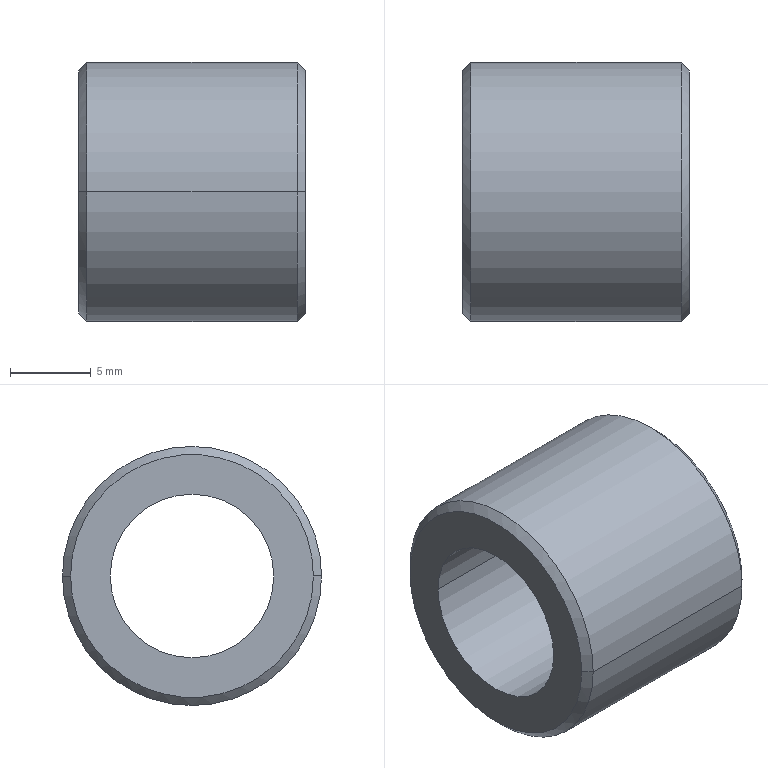Component | SolidWorks | ClampingArm2-1_A75-1 | 1 solid | 10 faces | box 14 x 16 x 16 mm | volume 1681 mm3 | cone 4 | cylinder 4 | plane 2 | commonest cylinder face diameters 10.1 x2 16 x2 | material Brass
build123d program:
from build123d import *

# Parameters (mm, degrees)
SKETCH1_R           = 8
SKETCH1_R_2         = 5.05
BOSS_EXTRUDE1_DEPTH = 7
CHAMFER1_SIZE       = 0.5


with BuildPart() as part:
    # Sketch1 → Boss-Extrude1 (new, symmetric)
    with BuildSketch(Plane(origin=(0, 0, 0), x_dir=(0, 0, -1), z_dir=(1, 0, 0))):
        Circle(SKETCH1_R)
        Circle(SKETCH1_R_2, mode=Mode.SUBTRACT)
    extrude(amount=BOSS_EXTRUDE1_DEPTH, both=True)

    # Chamfer1
    chamfer1_edges = [part.edges().sort_by_distance(p)[0] for p in [
        (-7, 0, 8),
        (7, 0, 8),
    ]]
    chamfer(chamfer1_edges, length=CHAMFER1_SIZE)


solid = part.part

# Placed as in the assembly
solid = solid.moved(Location((-22.051, 66.046, -22.5), (0, 0, 0)))
STEP:
#1=CARTESIAN_POINT('',(-0.5925,2.896,-0.8859));
#2=VERTEX_POINT('',#1);
#3=CARTESIAN_POINT('',(-0.5925,2.305,-0.8857));
#4=VERTEX_POINT('',#3);
#5=CARTESIAN_POINT('',(-0.5925,2.6,-0.8858));
#6=DIRECTION('',(1.,0.,-0.));
#7=DIRECTION('',(-0.,1.,-0.0003333));
#8=AXIS2_PLACEMENT_3D('',#5,#6,#7);
#9=CIRCLE('',#8,0.2953);
#10=EDGE_CURVE('',#2,#4,#9,.T.);
#11=ORIENTED_EDGE('',*,*,#10,.F.);
#12=CARTESIAN_POINT('',(-0.6122,2.915,-0.8859));
#13=VERTEX_POINT('',#12);
#14=CARTESIAN_POINT('',(-0.5925,2.896,-0.8859));
#15=DIRECTION('',(-0.7071,0.7071,-0.0002357));
#16=VECTOR('',#15,39.37);
#17=LINE('',#14,#16);
#18=EDGE_CURVE('',#2,#13,#17,.T.);
#19=ORIENTED_EDGE('',*,*,#18,.T.);
#20=CARTESIAN_POINT('',(-0.6122,2.285,-0.8857));
#21=VERTEX_POINT('',#20);
#22=CARTESIAN_POINT('',(-0.6122,2.6,-0.8858));
#23=DIRECTION('',(-1.,-0.,0.));
#24=DIRECTION('',(-0.,1.,-0.0003333));
#25=AXIS2_PLACEMENT_3D('',#22,#23,#24);
#26=CIRCLE('',#25,0.315);
#27=EDGE_CURVE('',#21,#13,#26,.T.);
#28=ORIENTED_EDGE('',*,*,#27,.F.);
#29=CARTESIAN_POINT('',(-0.5925,2.305,-0.8857));
#30=DIRECTION('',(-0.7071,-0.7071,0.0002357));
#31=VECTOR('',#30,39.37);
#32=LINE('',#29,#31);
#33=EDGE_CURVE('',#4,#21,#32,.T.);
#34=ORIENTED_EDGE('',*,*,#33,.F.);
#35=EDGE_LOOP('',(#11,#19,#28,#34));
#36=FACE_OUTER_BOUND('',#35,.T.);
#37=CARTESIAN_POINT('',(-0.5925,2.6,-0.8858));
#38=DIRECTION('',(-1.,-0.,0.));
#39=DIRECTION('',(0.,-1.,0.0003333));
#40=AXIS2_PLACEMENT_3D('',#37,#38,#39);
#41=CONICAL_SURFACE('',#40,0.2953,0.7854);
#42=ADVANCED_FACE('',(#36),#41,.T.);
#43=CARTESIAN_POINT('',(-1.144,2.305,-0.8857));
#44=VERTEX_POINT('',#43);
#45=CARTESIAN_POINT('',(-1.144,2.896,-0.8859));
#46=VERTEX_POINT('',#45);
#47=CARTESIAN_POINT('',(-1.144,2.6,-0.8858));
#48=DIRECTION('',(-1.,-0.,0.));
#49=DIRECTION('',(-0.,1.,-0.0003333));
#50=AXIS2_PLACEMENT_3D('',#47,#48,#49);
#51=CIRCLE('',#50,0.2953);
#52=EDGE_CURVE('',#44,#46,#51,.T.);
#53=ORIENTED_EDGE('',*,*,#52,.F.);
#54=CARTESIAN_POINT('',(-1.124,2.285,-0.8857));
#55=VERTEX_POINT('',#54);
#56=CARTESIAN_POINT('',(-1.124,2.285,-0.8857));
#57=DIRECTION('',(0.7071,-0.7071,0.0002357));
#58=VECTOR('',#57,39.37);
#59=LINE('',#56,#58);
#60=EDGE_CURVE('',#44,#55,#59,.T.);
#61=ORIENTED_EDGE('',*,*,#60,.T.);
#62=CARTESIAN_POINT('',(-1.124,2.915,-0.8859));
#63=VERTEX_POINT('',#62);
#64=CARTESIAN_POINT('',(-1.124,2.6,-0.8858));
#65=DIRECTION('',(1.,0.,-0.));
#66=DIRECTION('',(-0.,1.,-0.0003333));
#67=AXIS2_PLACEMENT_3D('',#64,#65,#66);
#68=CIRCLE('',#67,0.315);
#69=EDGE_CURVE('',#63,#55,#68,.T.);
#70=ORIENTED_EDGE('',*,*,#69,.F.);
#71=CARTESIAN_POINT('',(-1.124,2.915,-0.8859));
#72=DIRECTION('',(0.7071,0.7071,-0.0002357));
#73=VECTOR('',#72,39.37);
#74=LINE('',#71,#73);
#75=EDGE_CURVE('',#46,#63,#74,.T.);
#76=ORIENTED_EDGE('',*,*,#75,.F.);
#77=EDGE_LOOP('',(#53,#61,#70,#76));
#78=FACE_OUTER_BOUND('',#77,.T.);
#79=CARTESIAN_POINT('',(-1.124,2.6,-0.8858));
#80=DIRECTION('',(1.,0.,-0.));
#81=DIRECTION('',(-0.,1.,-0.0003333));
#82=AXIS2_PLACEMENT_3D('',#79,#80,#81);
#83=CONICAL_SURFACE('',#82,0.315,0.7854);
#84=ADVANCED_FACE('',(#78),#83,.T.);
#85=CARTESIAN_POINT('',(-0.5925,2.401,-0.8858));
#86=VERTEX_POINT('',#85);
#87=CARTESIAN_POINT('',(-0.5925,2.799,-0.8859));
#88=VERTEX_POINT('',#87);
#89=CARTESIAN_POINT('',(-0.5925,2.6,-0.8858));
#90=DIRECTION('',(1.,0.,-0.));
#91=DIRECTION('',(-0.,1.,-0.0003333));
#92=AXIS2_PLACEMENT_3D('',#89,#90,#91);
#93=CIRCLE('',#92,0.1988);
#94=EDGE_CURVE('',#86,#88,#93,.T.);
#95=ORIENTED_EDGE('',*,*,#94,.T.);
#96=CARTESIAN_POINT('',(-1.144,2.799,-0.8859));
#97=VERTEX_POINT('',#96);
#98=CARTESIAN_POINT('',(-0.5925,2.799,-0.8859));
#99=DIRECTION('',(-1.,-0.,0.));
#100=VECTOR('',#99,39.37);
#101=LINE('',#98,#100);
#102=EDGE_CURVE('',#88,#97,#101,.T.);
#103=ORIENTED_EDGE('',*,*,#102,.T.);
#104=CARTESIAN_POINT('',(-1.144,2.401,-0.8858));
#105=VERTEX_POINT('',#104);
#106=CARTESIAN_POINT('',(-1.144,2.6,-0.8858));
#107=DIRECTION('',(1.,0.,-0.));
#108=DIRECTION('',(0.,1.,-0.0003333));
#109=AXIS2_PLACEMENT_3D('',#106,#107,#108);
#110=CIRCLE('',#109,0.1988);
#111=EDGE_CURVE('',#105,#97,#110,.T.);
#112=ORIENTED_EDGE('',*,*,#111,.F.);
#113=CARTESIAN_POINT('',(-0.5925,2.401,-0.8858));
#114=DIRECTION('',(-1.,-0.,0.));
#115=VECTOR('',#114,39.37);
#116=LINE('',#113,#115);
#117=EDGE_CURVE('',#86,#105,#116,.T.);
#118=ORIENTED_EDGE('',*,*,#117,.F.);
#119=EDGE_LOOP('',(#95,#103,#112,#118));
#120=FACE_OUTER_BOUND('',#119,.T.);
#121=CARTESIAN_POINT('',(-0.5925,2.6,-0.8858));
#122=DIRECTION('',(-1.,-0.,0.));
#123=DIRECTION('',(0.,-1.,0.0003333));
#124=AXIS2_PLACEMENT_3D('',#121,#122,#123);
#125=CYLINDRICAL_SURFACE('',#124,0.1988);
#126=ADVANCED_FACE('',(#120),#125,.F.);
#127=ORIENTED_EDGE('',*,*,#27,.T.);
#128=CARTESIAN_POINT('',(-0.5925,2.915,-0.8859));
#129=DIRECTION('',(-1.,-0.,0.));
#130=VECTOR('',#129,39.37);
#131=LINE('',#128,#130);
#132=EDGE_CURVE('',#13,#63,#131,.T.);
#133=ORIENTED_EDGE('',*,*,#132,.T.);
#134=ORIENTED_EDGE('',*,*,#69,.T.);
#135=CARTESIAN_POINT('',(-0.5925,2.285,-0.8857));
#136=DIRECTION('',(-1.,-0.,0.));
#137=VECTOR('',#136,39.37);
#138=LINE('',#135,#137);
#139=EDGE_CURVE('',#21,#55,#138,.T.);
#140=ORIENTED_EDGE('',*,*,#139,.F.);
#141=EDGE_LOOP('',(#127,#133,#134,#140));
#142=FACE_OUTER_BOUND('',#141,.T.);
#143=CARTESIAN_POINT('',(-0.5925,2.6,-0.8858));
#144=DIRECTION('',(-1.,-0.,0.));
#145=DIRECTION('',(0.,-1.,0.0003333));
#146=AXIS2_PLACEMENT_3D('',#143,#144,#145);
#147=CYLINDRICAL_SURFACE('',#146,0.315);
#148=ADVANCED_FACE('',(#142),#147,.T.);
#149=CARTESIAN_POINT('',(-0.5925,2.6,-0.8858));
#150=DIRECTION('',(1.,0.,-0.));
#151=DIRECTION('',(-0.,1.,-0.0003333));
#152=AXIS2_PLACEMENT_3D('',#149,#150,#151);
#153=CIRCLE('',#152,0.2953);
#154=EDGE_CURVE('',#4,#2,#153,.T.);
#155=ORIENTED_EDGE('',*,*,#154,.T.);
#156=ORIENTED_EDGE('',*,*,#10,.T.);
#157=EDGE_LOOP('',(#155,#156));
#158=FACE_OUTER_BOUND('',#157,.T.);
#159=ORIENTED_EDGE('',*,*,#94,.F.);
#160=CARTESIAN_POINT('',(-0.5925,2.6,-0.8858));
#161=DIRECTION('',(1.,0.,-0.));
#162=DIRECTION('',(-0.,1.,-0.0003333));
#163=AXIS2_PLACEMENT_3D('',#160,#161,#162);
#164=CIRCLE('',#163,0.1988);
#165=EDGE_CURVE('',#88,#86,#164,.T.);
#166=ORIENTED_EDGE('',*,*,#165,.F.);
#167=EDGE_LOOP('',(#159,#166));
#168=FACE_BOUND('',#167,.T.);
#169=CARTESIAN_POINT('',(-0.5925,2.6,-0.8858));
#170=DIRECTION('',(1.,0.,-0.));
#171=DIRECTION('',(-0.,1.,-0.0003333));
#172=AXIS2_PLACEMENT_3D('',#169,#170,#171);
#173=PLANE('',#172);
#174=ADVANCED_FACE('',(#158,#168),#173,.T.);
#175=CARTESIAN_POINT('',(-1.144,2.6,-0.8858));
#176=DIRECTION('',(-1.,-0.,0.));
#177=DIRECTION('',(-0.,1.,-0.0003333));
#178=AXIS2_PLACEMENT_3D('',#175,#176,#177);
#179=CIRCLE('',#178,0.2953);
#180=EDGE_CURVE('',#46,#44,#179,.T.);
#181=ORIENTED_EDGE('',*,*,#180,.T.);
#182=ORIENTED_EDGE('',*,*,#52,.T.);
#183=EDGE_LOOP('',(#181,#182));
#184=FACE_OUTER_BOUND('',#183,.T.);
#185=ORIENTED_EDGE('',*,*,#111,.T.);
#186=CARTESIAN_POINT('',(-1.144,2.6,-0.8858));
#187=DIRECTION('',(1.,0.,-0.));
#188=DIRECTION('',(0.,1.,-0.0003333));
#189=AXIS2_PLACEMENT_3D('',#186,#187,#188);
#190=CIRCLE('',#189,0.1988);
#191=EDGE_CURVE('',#97,#105,#190,.T.);
#192=ORIENTED_EDGE('',*,*,#191,.T.);
#193=EDGE_LOOP('',(#185,#192));
#194=FACE_BOUND('',#193,.T.);
#195=CARTESIAN_POINT('',(-1.144,2.6,-0.8858));
#196=DIRECTION('',(1.,0.,-0.));
#197=DIRECTION('',(-0.,1.,-0.0003333));
#198=AXIS2_PLACEMENT_3D('',#195,#196,#197);
#199=PLANE('',#198);
#200=ADVANCED_FACE('',(#184,#194),#199,.F.);
#201=ORIENTED_EDGE('',*,*,#132,.F.);
#202=CARTESIAN_POINT('',(-0.6122,2.6,-0.8858));
#203=DIRECTION('',(-1.,-0.,0.));
#204=DIRECTION('',(-0.,1.,-0.0003333));
#205=AXIS2_PLACEMENT_3D('',#202,#203,#204);
#206=CIRCLE('',#205,0.315);
#207=EDGE_CURVE('',#13,#21,#206,.T.);
#208=ORIENTED_EDGE('',*,*,#207,.T.);
#209=ORIENTED_EDGE('',*,*,#139,.T.);
#210=CARTESIAN_POINT('',(-1.124,2.6,-0.8858));
#211=DIRECTION('',(1.,0.,-0.));
#212=DIRECTION('',(-0.,1.,-0.0003333));
#213=AXIS2_PLACEMENT_3D('',#210,#211,#212);
#214=CIRCLE('',#213,0.315);
#215=EDGE_CURVE('',#55,#63,#214,.T.);
#216=ORIENTED_EDGE('',*,*,#215,.T.);
#217=EDGE_LOOP('',(#201,#208,#209,#216));
#218=FACE_OUTER_BOUND('',#217,.T.);
#219=CARTESIAN_POINT('',(-0.5925,2.6,-0.8858));
#220=DIRECTION('',(-1.,-0.,0.));
#221=DIRECTION('',(0.,-1.,0.0003333));
#222=AXIS2_PLACEMENT_3D('',#219,#220,#221);
#223=CYLINDRICAL_SURFACE('',#222,0.315);
#224=ADVANCED_FACE('',(#218),#223,.T.);
#225=ORIENTED_EDGE('',*,*,#102,.F.);
#226=ORIENTED_EDGE('',*,*,#165,.T.);
#227=ORIENTED_EDGE('',*,*,#117,.T.);
#228=ORIENTED_EDGE('',*,*,#191,.F.);
#229=EDGE_LOOP('',(#225,#226,#227,#228));
#230=FACE_OUTER_BOUND('',#229,.T.);
#231=CARTESIAN_POINT('',(-0.5925,2.6,-0.8858));
#232=DIRECTION('',(-1.,-0.,0.));
#233=DIRECTION('',(0.,-1.,0.0003333));
#234=AXIS2_PLACEMENT_3D('',#231,#232,#233);
#235=CYLINDRICAL_SURFACE('',#234,0.1988);
#236=ADVANCED_FACE('',(#230),#235,.F.);
#237=ORIENTED_EDGE('',*,*,#60,.F.);
#238=ORIENTED_EDGE('',*,*,#180,.F.);
#239=ORIENTED_EDGE('',*,*,#75,.T.);
#240=ORIENTED_EDGE('',*,*,#215,.F.);
#241=EDGE_LOOP('',(#237,#238,#239,#240));
#242=FACE_OUTER_BOUND('',#241,.T.);
#243=CARTESIAN_POINT('',(-1.124,2.6,-0.8858));
#244=DIRECTION('',(1.,0.,-0.));
#245=DIRECTION('',(-0.,1.,-0.0003333));
#246=AXIS2_PLACEMENT_3D('',#243,#244,#245);
#247=CONICAL_SURFACE('',#246,0.315,0.7854);
#248=ADVANCED_FACE('',(#242),#247,.T.);
#249=ORIENTED_EDGE('',*,*,#18,.F.);
#250=ORIENTED_EDGE('',*,*,#154,.F.);
#251=ORIENTED_EDGE('',*,*,#33,.T.);
#252=ORIENTED_EDGE('',*,*,#207,.F.);
#253=EDGE_LOOP('',(#249,#250,#251,#252));
#254=FACE_OUTER_BOUND('',#253,.T.);
#255=CARTESIAN_POINT('',(-0.5925,2.6,-0.8858));
#256=DIRECTION('',(-1.,-0.,0.));
#257=DIRECTION('',(0.,-1.,0.0003333));
#258=AXIS2_PLACEMENT_3D('',#255,#256,#257);
#259=CONICAL_SURFACE('',#258,0.2953,0.7854);
#260=ADVANCED_FACE('',(#254),#259,.T.);
#261=CLOSED_SHELL('',(#42,#84,#126,#148,#174,#200,#224,#236,#248,#260));
#262=MANIFOLD_SOLID_BREP('',#261);
#263=CARTESIAN_POINT('',(0.,0.,0.));
#264=DIRECTION('',(0.,0.,1.));
#265=DIRECTION('',(1.,0.,0.));
#266=AXIS2_PLACEMENT_3D('',#263,#264,#265);
#267=(LENGTH_UNIT()NAMED_UNIT(*)SI_UNIT($,.METRE.));
#268=LENGTH_MEASURE_WITH_UNIT(LENGTH_MEASURE(0.0254),#267);
#269=DIMENSIONAL_EXPONENTS(1.,0.,0.,0.,0.,0.,0.);
#270=(CONVERSION_BASED_UNIT('',#268)LENGTH_UNIT()NAMED_UNIT(#269));
#271=UNCERTAINTY_MEASURE_WITH_UNIT(LENGTH_MEASURE(0.00001),#270,'','');
#272=(NAMED_UNIT(*)PLANE_ANGLE_UNIT()SI_UNIT($,.RADIAN.));
#273=(NAMED_UNIT(*)SI_UNIT($,.STERADIAN.)SOLID_ANGLE_UNIT());
#274=(GEOMETRIC_REPRESENTATION_CONTEXT(3)GLOBAL_UNCERTAINTY_ASSIGNED_CONTEXT((#271))GLOBAL_UNIT_ASSIGNED_CONTEXT((#270,#272,#273))REPRESENTATION_CONTEXT('',''));
#275=ADVANCED_BREP_SHAPE_REPRESENTATION('',(#262,#266),#274);
#276=COLOUR_RGB('',0.7922,0.8196,0.9333);
#277=FILL_AREA_STYLE_COLOUR('',#276);
#278=FILL_AREA_STYLE('',(#277));
#279=SURFACE_STYLE_FILL_AREA(#278);
#280=SURFACE_SIDE_STYLE('',(#279));
#281=SURFACE_STYLE_USAGE(.BOTH.,#280);
#282=PRESENTATION_STYLE_ASSIGNMENT((#281));
#283=STYLED_ITEM('',(#282),#262);
#284=(LENGTH_UNIT()NAMED_UNIT(*)SI_UNIT($,.METRE.));
#285=LENGTH_MEASURE_WITH_UNIT(LENGTH_MEASURE(0.0254),#284);
#286=DIMENSIONAL_EXPONENTS(1.,0.,0.,0.,0.,0.,0.);
#287=(CONVERSION_BASED_UNIT('',#285)LENGTH_UNIT()NAMED_UNIT(#286));
#288=UNCERTAINTY_MEASURE_WITH_UNIT(LENGTH_MEASURE(0.00001),#287,'','');
#289=(NAMED_UNIT(*)PLANE_ANGLE_UNIT()SI_UNIT($,.RADIAN.));
#290=(NAMED_UNIT(*)SI_UNIT($,.STERADIAN.)SOLID_ANGLE_UNIT());
#291=(GEOMETRIC_REPRESENTATION_CONTEXT(3)GLOBAL_UNCERTAINTY_ASSIGNED_CONTEXT((#288))GLOBAL_UNIT_ASSIGNED_CONTEXT((#287,#289,#290))REPRESENTATION_CONTEXT('',''));
#292=MECHANICAL_DESIGN_GEOMETRIC_PRESENTATION_REPRESENTATION('',(#283),#291);
#293=PRESENTATION_LAYER_ASSIGNMENT('','',(#283));